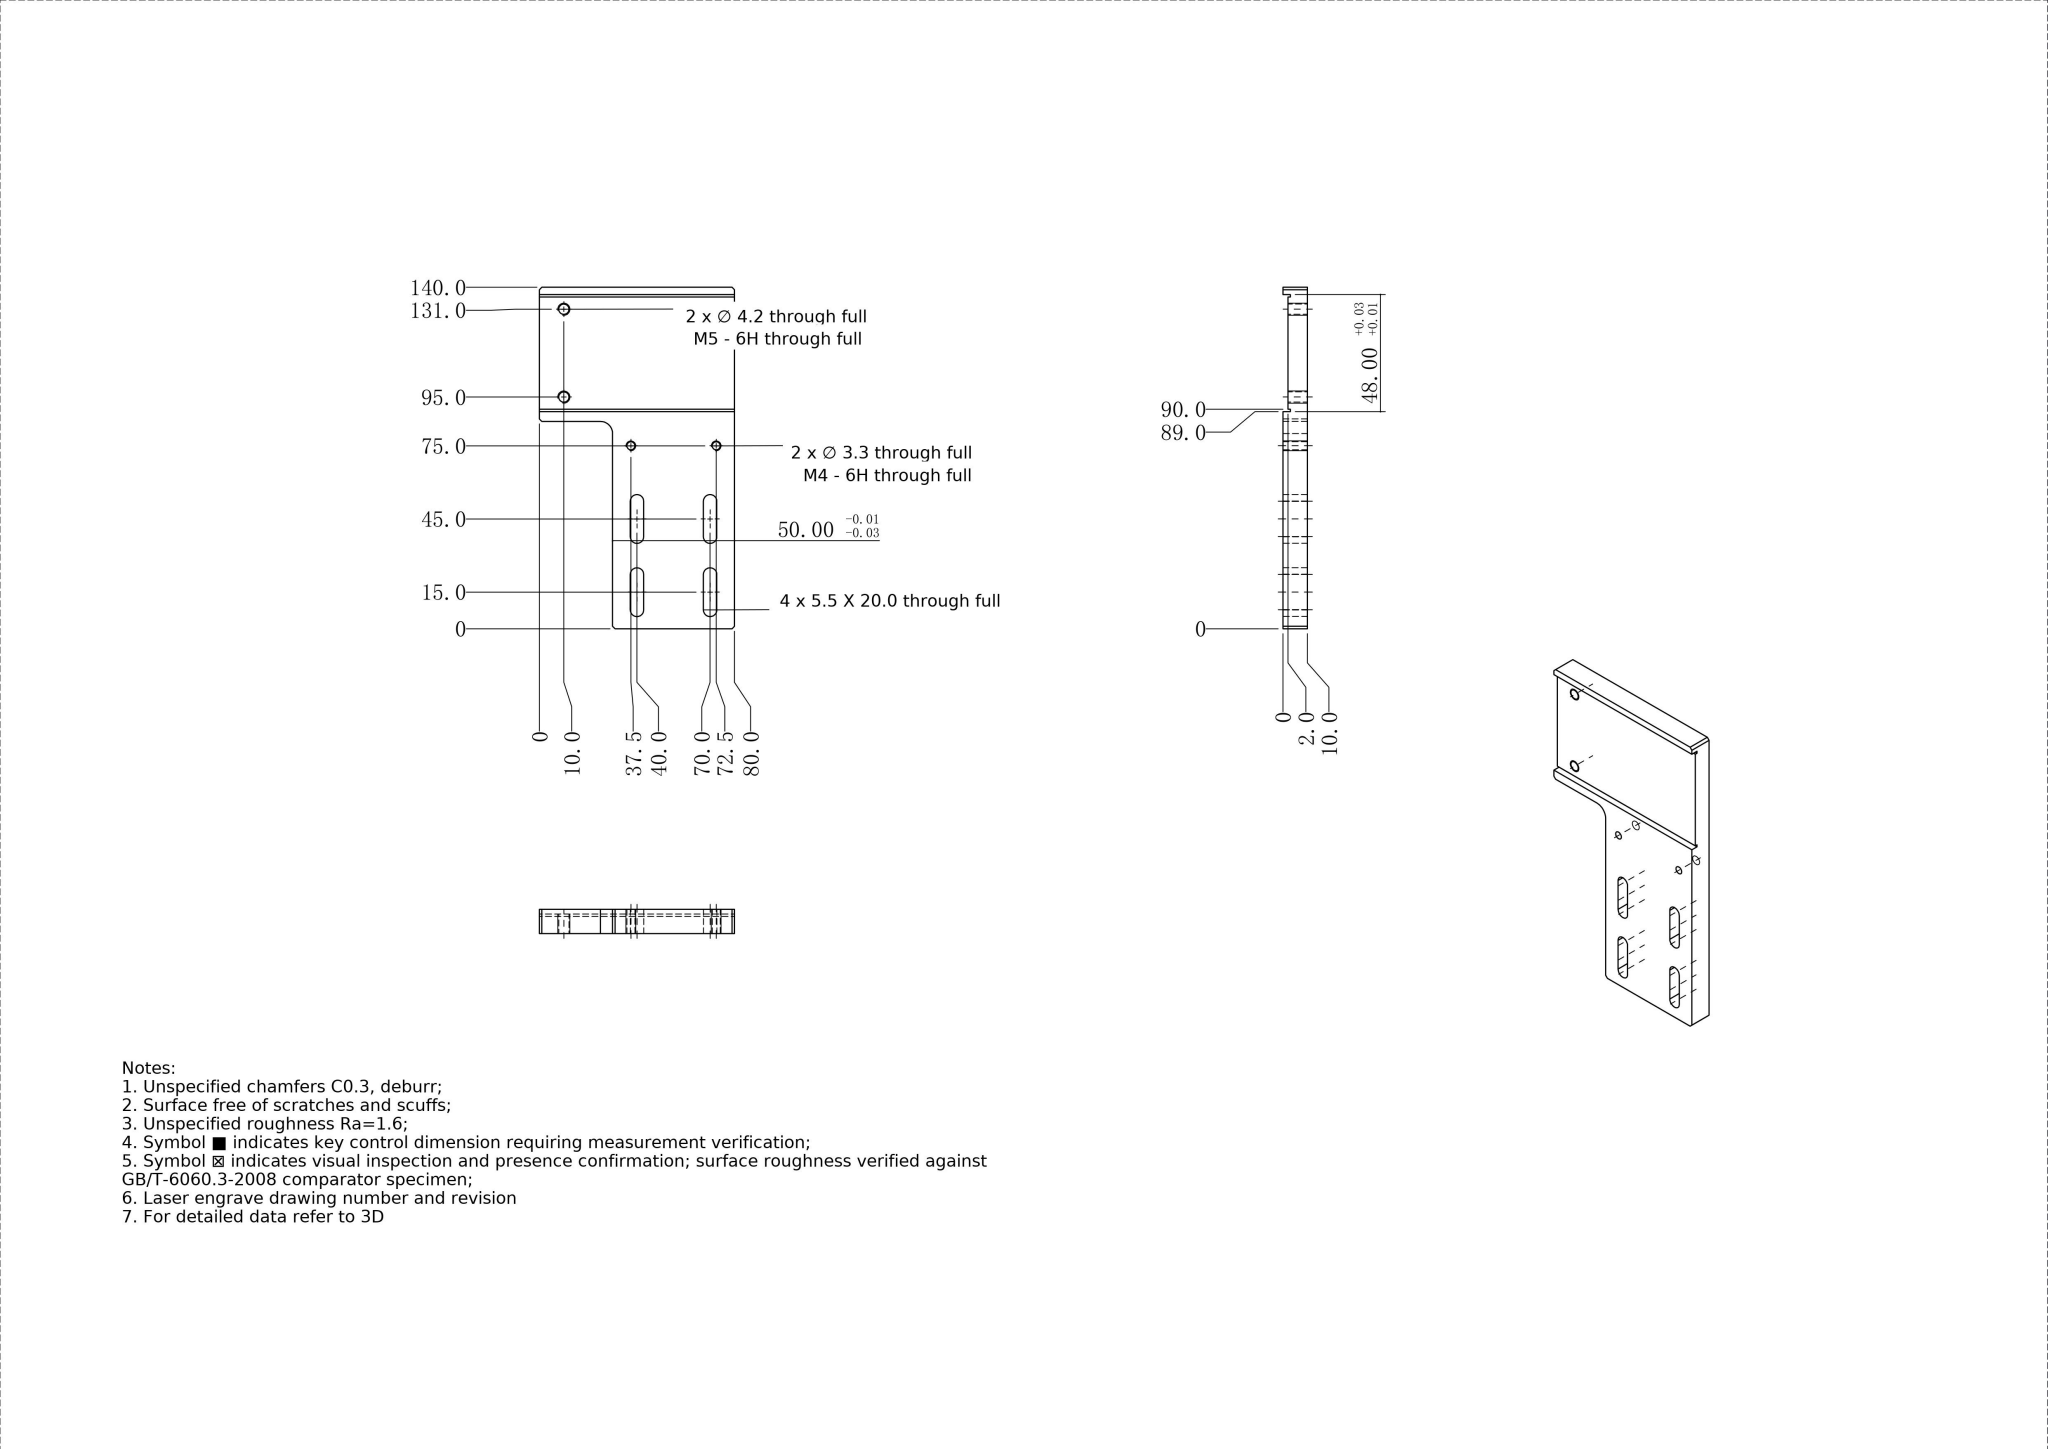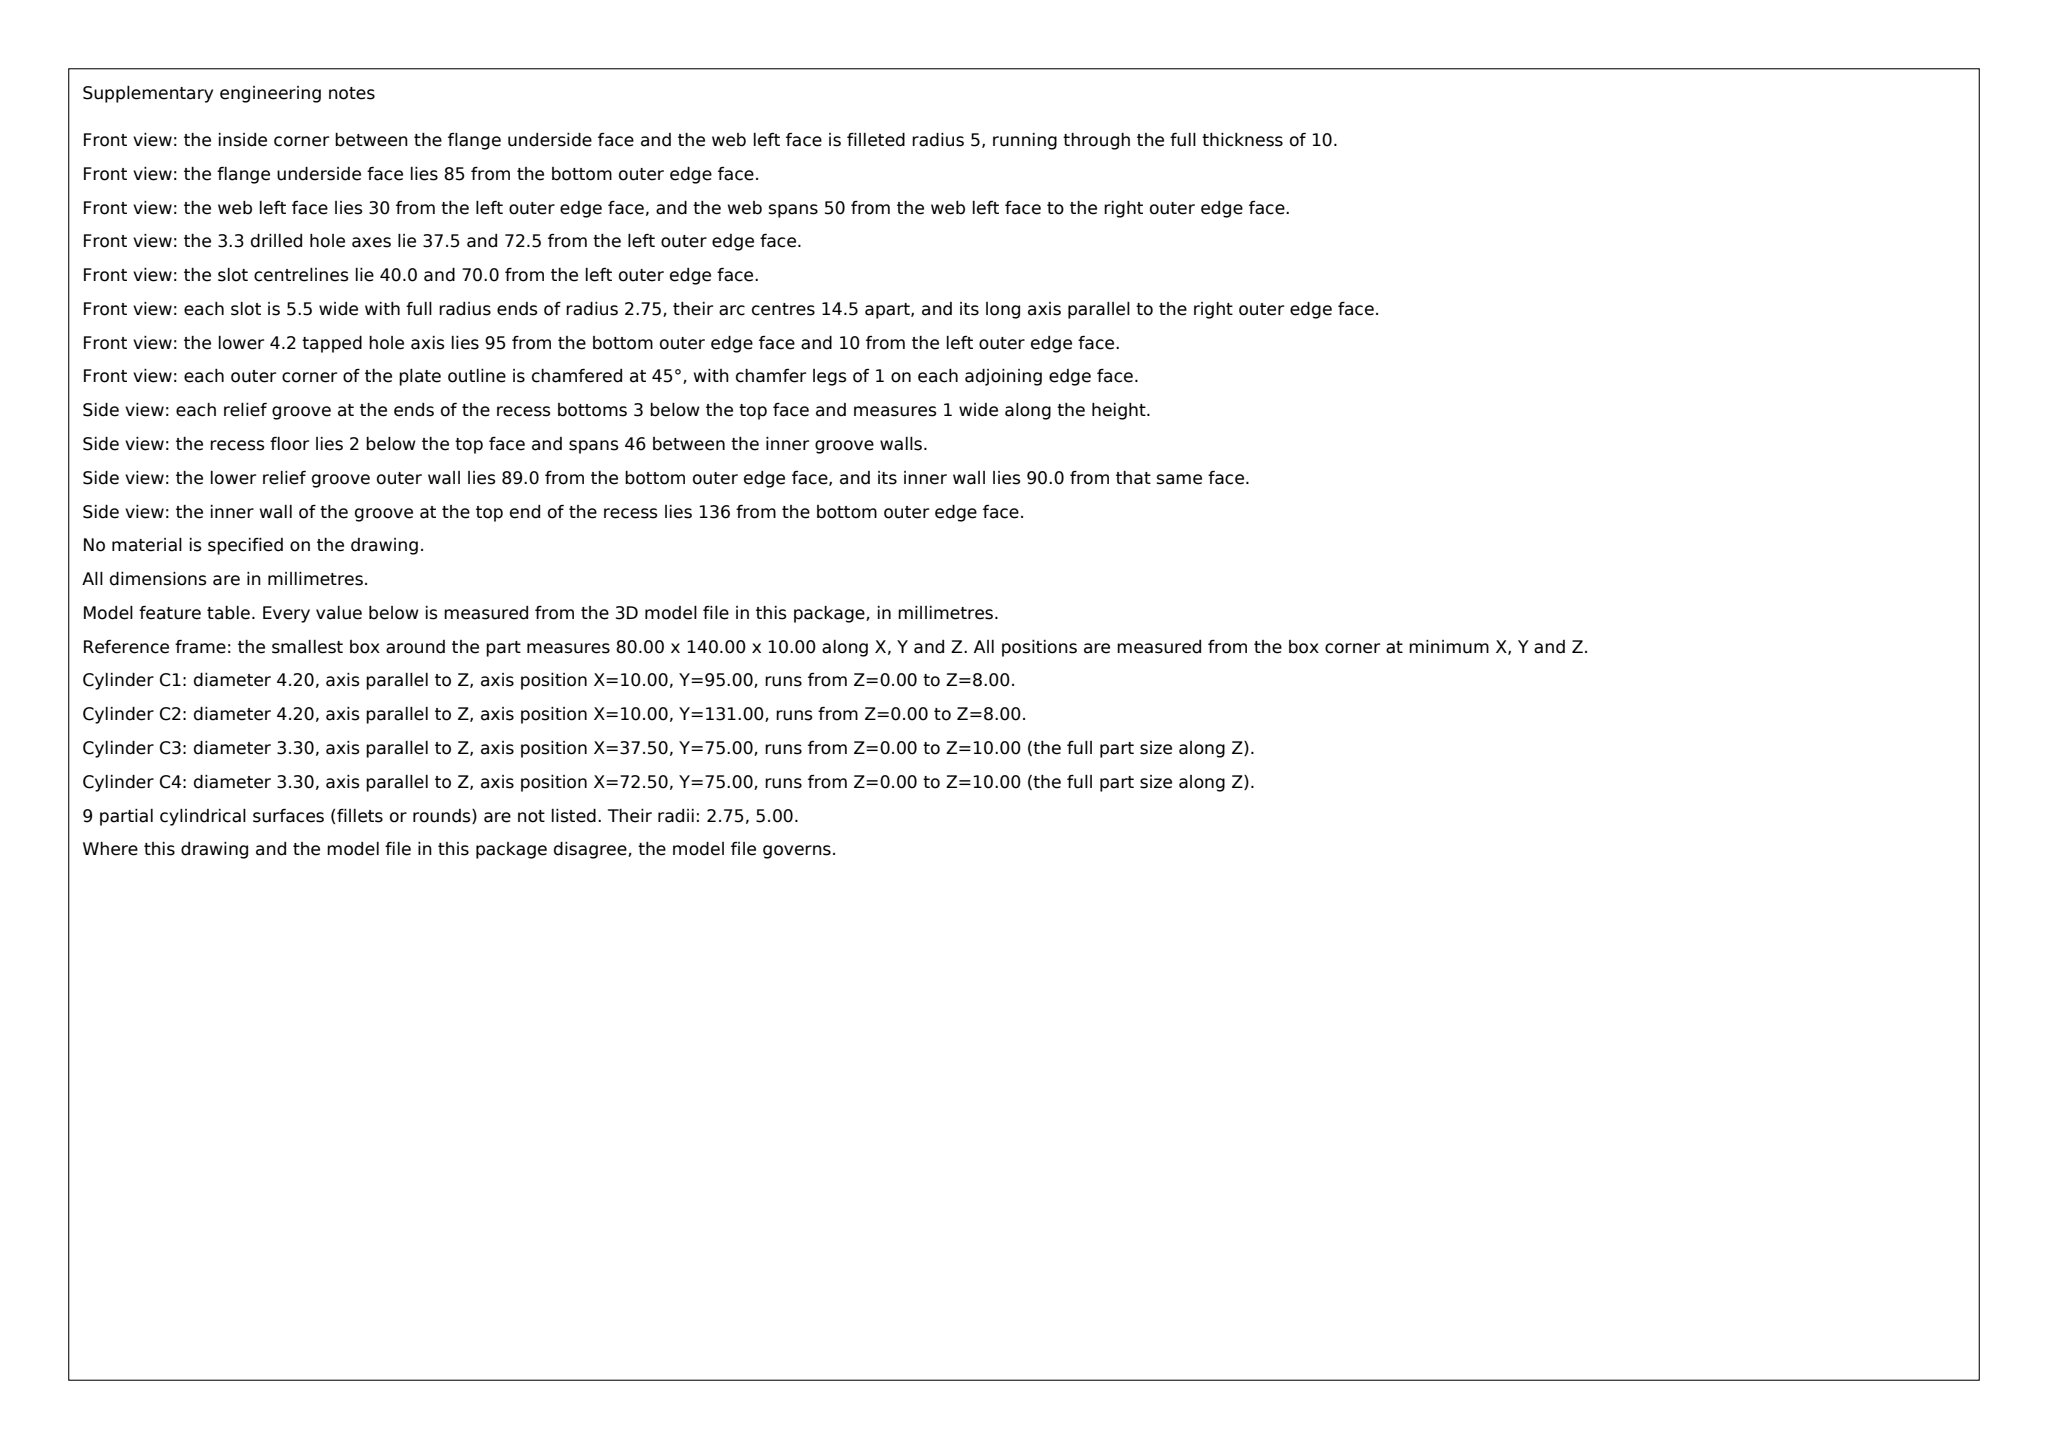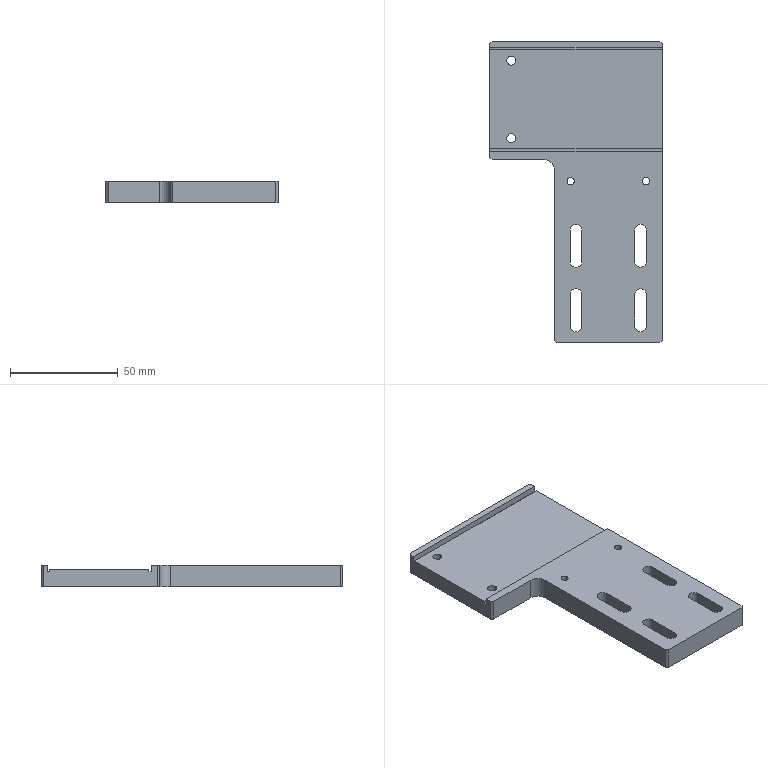Part | SolidWorks | mm | 1 solid | 46 faces | box 80 x 140 x 10 mm | volume 74156 mm3 | plane 29 | cylinder 17 | commonest cylinder face diameters 5.5 x8 4.2 x4 3.3 x4 10 x1